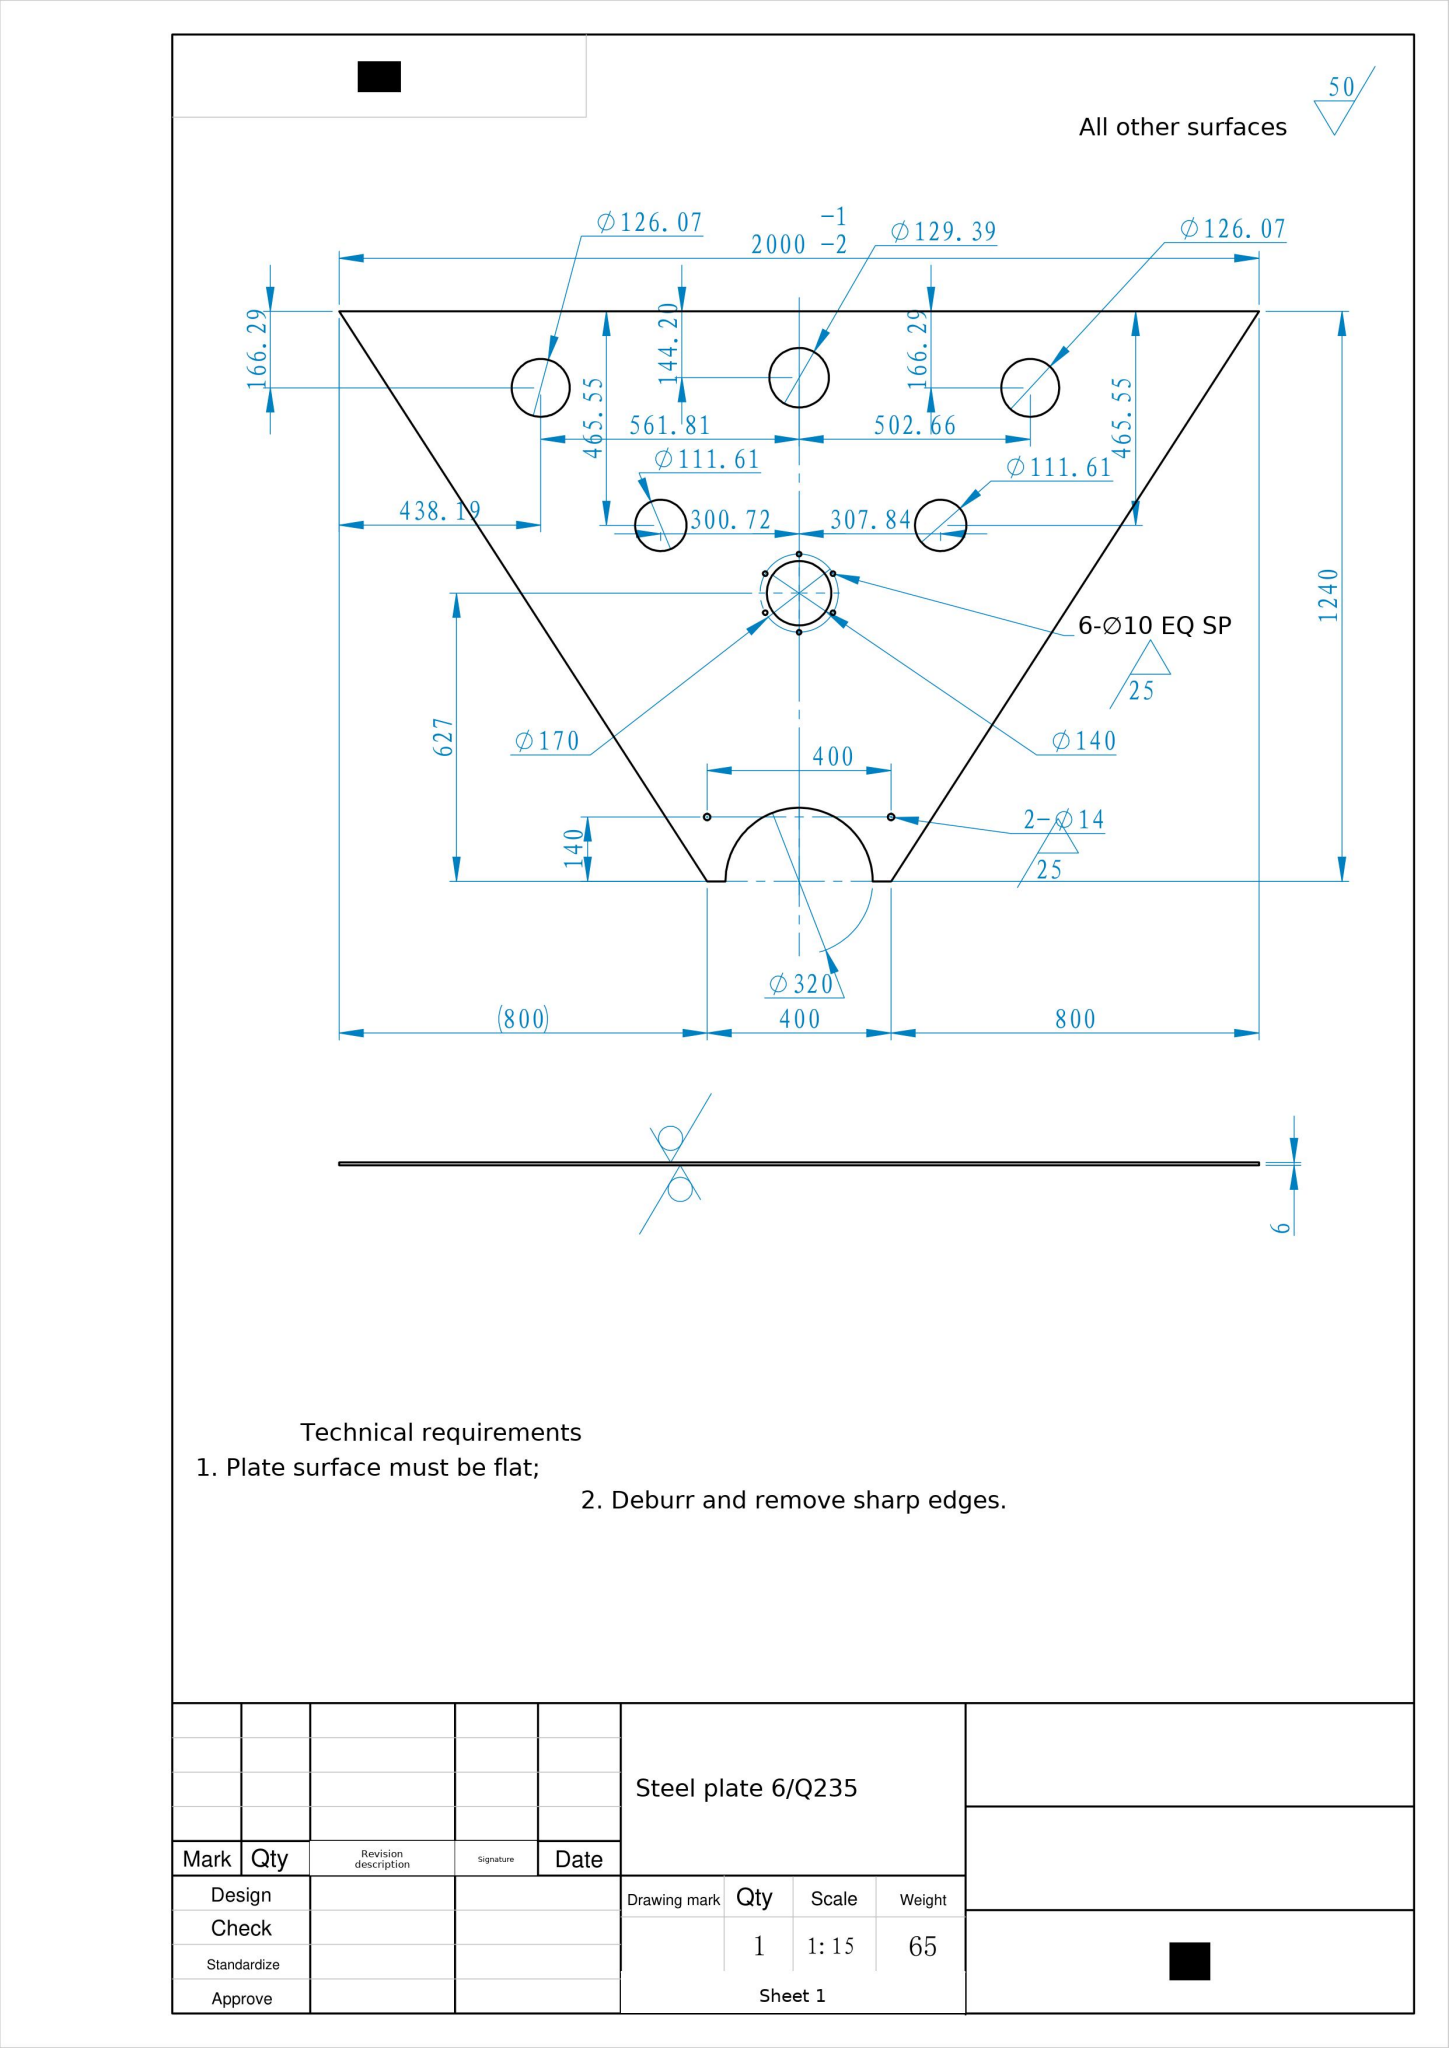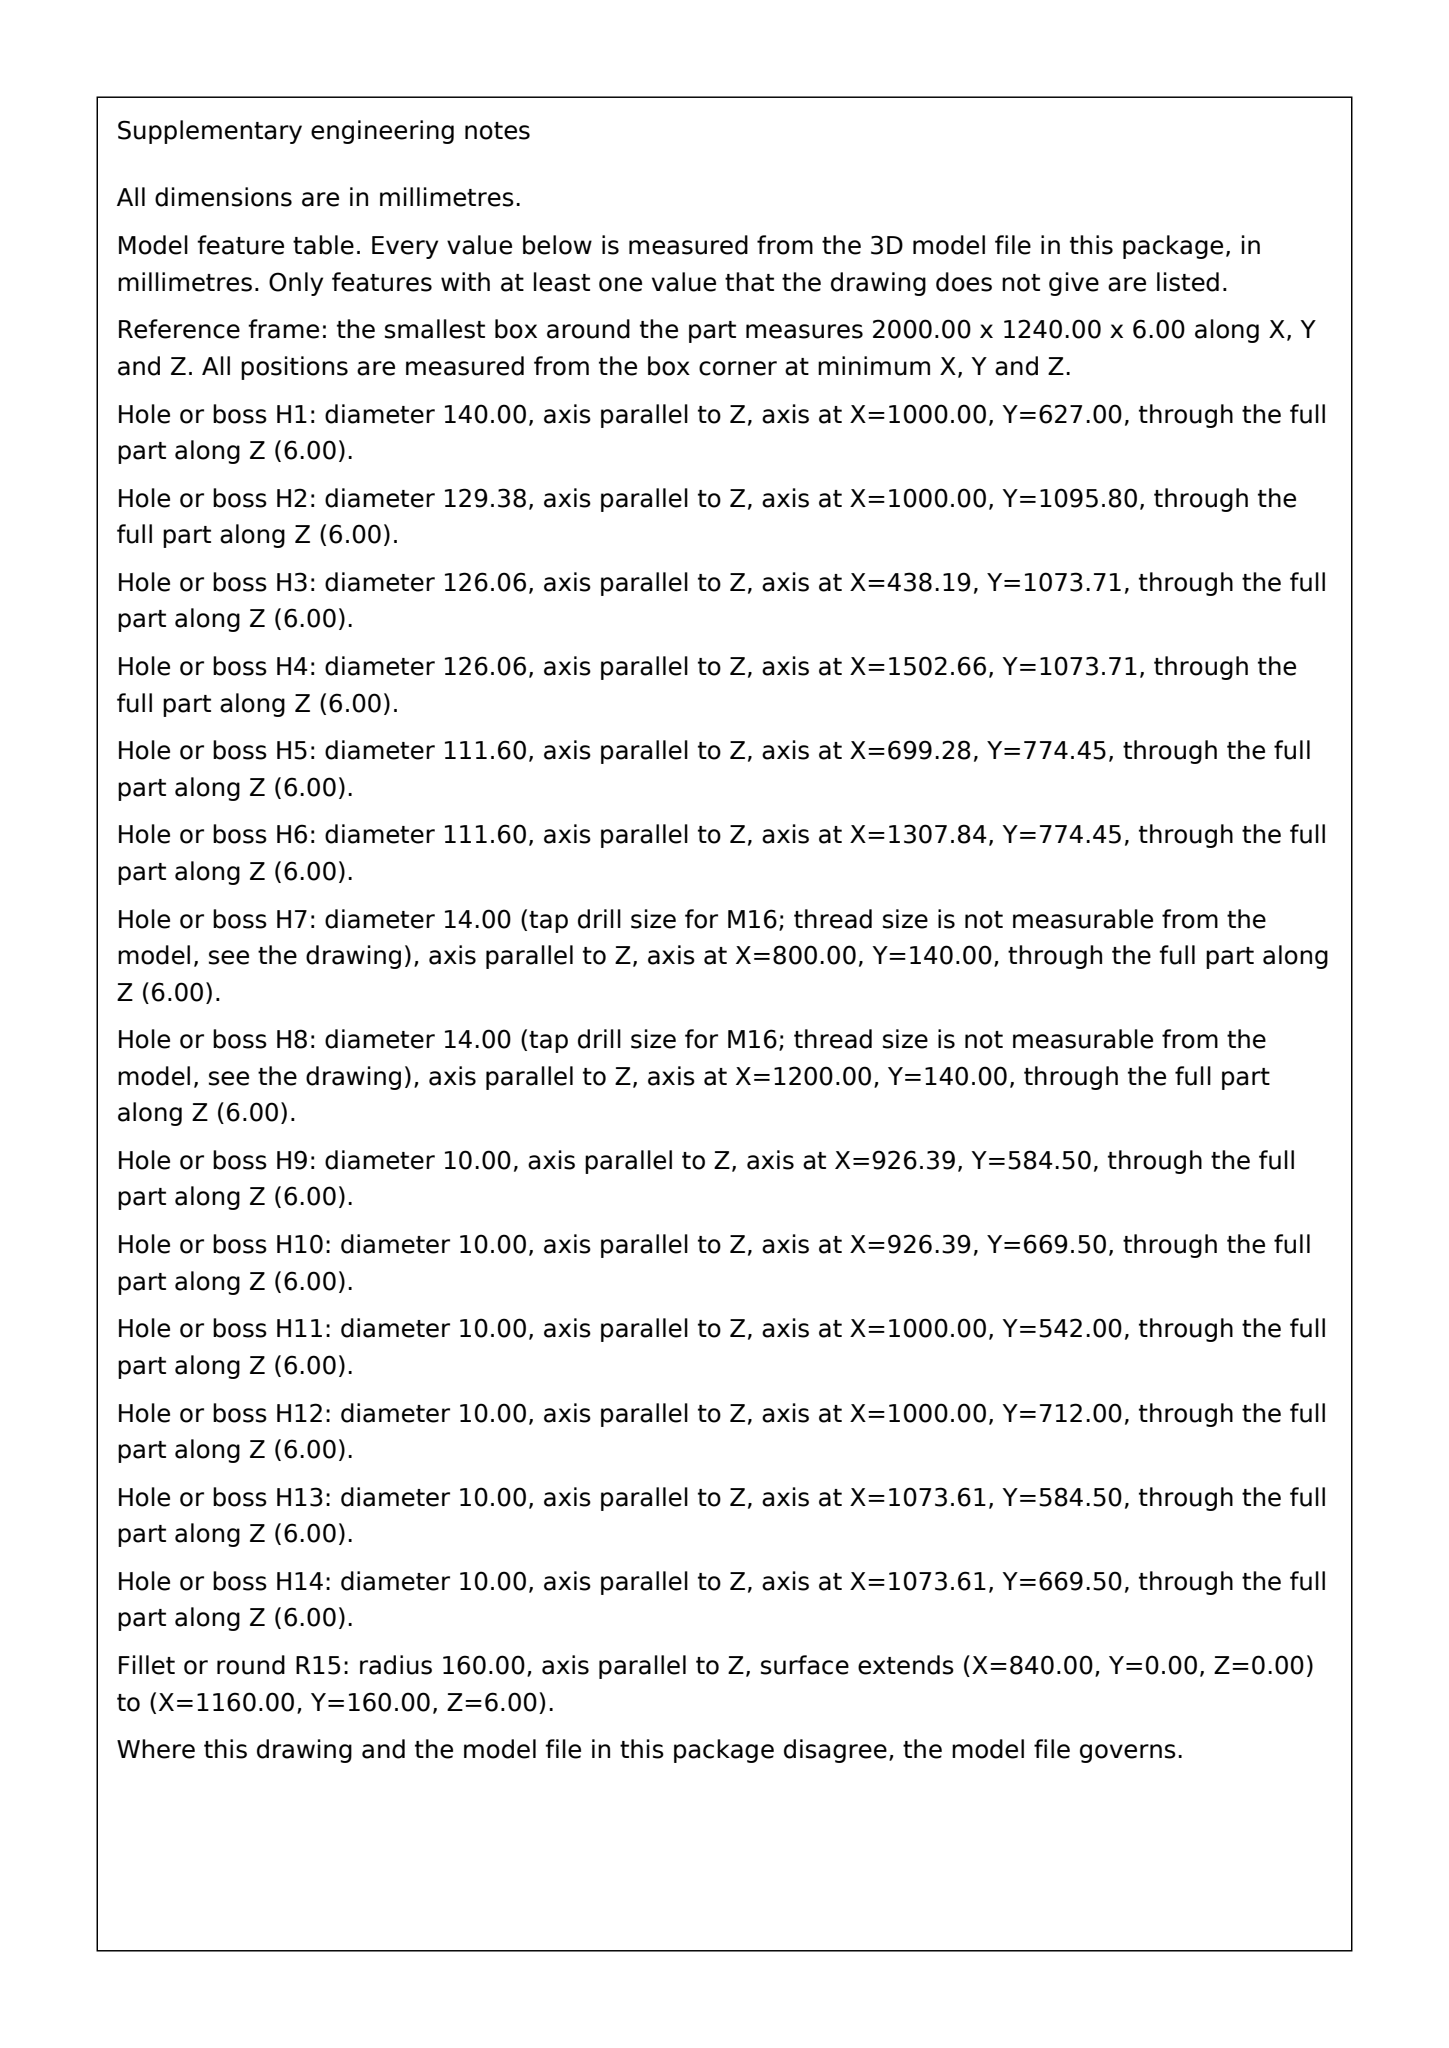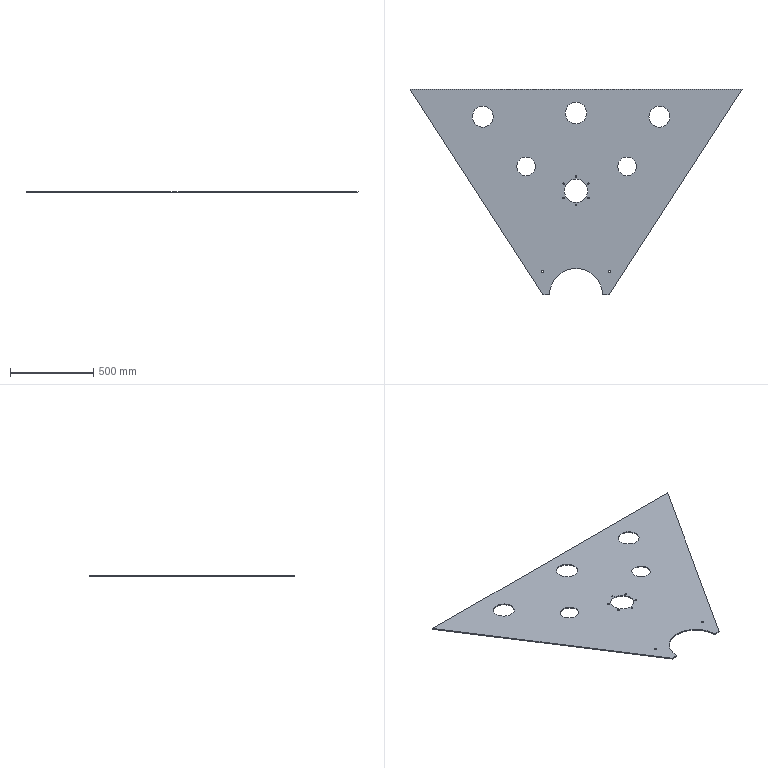Part | SolidWorks | mm | material Steel plate 6/Q235 | 1 solid | 36 faces | box 2000 x 1240 x 6 mm | volume 8243608 mm3 | cylinder 29 | plane 7 | commonest cylinder face diameters 10 x12 126.069 x4 111.609 x4 14 x4 129.385 x2 140 x2 320 x1